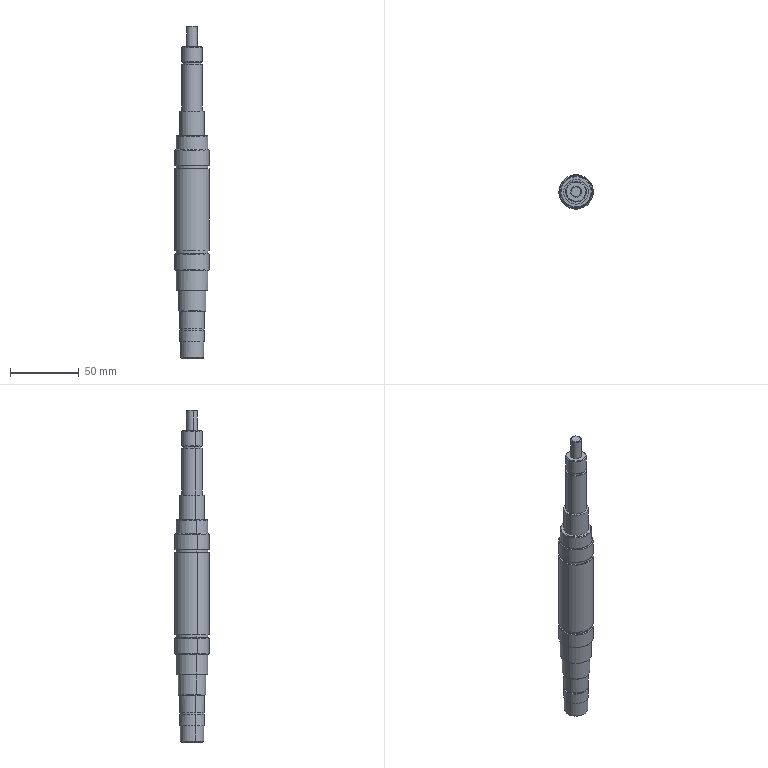Component | SolidWorks | BladeDriveAxis0-2 | 1 solid | 90 faces | box 25 x 25 x 242 mm | volume 78824 mm3 | cylinder 41 | plane 30 | cone 19 | commonest cylinder face diameters 23 x8 18 x6 25 x6 5 x5 15 x4 17 x4 20 x2 13 x2
build123d program:
from build123d import *

# Parameters (mm, degrees)
CUT_EXTRUDE1_2_START = 9.25
CUT_EXTRUDE1_2_DEPTH = 10
CUT_EXTRUDE2_START   = 5.5
CUT_EXTRUDE2_DEPTH   = 10
CUT_EXTRUDE3_START   = 5.8
CUT_EXTRUDE3_DEPTH   = 10
CUT_EXTRUDE1_START   = 9.25
CUT_EXTRUDE1_DEPTH   = 10


with BuildPart() as part:
    # Sketch1_2 → Revolve1 (revolve)
    with BuildSketch(Plane.XY, mode=Mode.PRIVATE) as revolve1_sk:
        Polygon((-96, 8.5), (-96, 9), (-87.7, 9), (-87.7, 8.5), (-86.6, 8.5), (-86.6, 9), (-74, 9), (-74, 9.5), (-73.5, 10), (-59, 10), (-59, 11), (-58.5, 11.5), (-44, 11.5), (-44, 12), (-43.5, 12.5), (-32.5, 12.5), (-32, 12), (-32, 11.5), (-30, 11.5), (-30, 12.5), (30, 12.5), (30, 11.5), (32, 11.5), (32, 12), (32.5, 12.5), (43.5, 12.5), (44, 12), (44, 11.5), (53.5, 11.5), (54, 11), (54, 9), (72, 9), (72, 7.5), (106, 7.5), (106, 6.5), (107.5, 6.5), (107.5, 7), (108, 7.5), (118.5, 7.5), (119, 7), (119, 4), (133.5, 4), (134, 3.5), (134, 0), (-108, 0), (-108, 8), (-107.5, 8.5), align=None)
    revolve(revolve1_sk.sketch.rotate(Axis((-108, 0, 0), (1, 0, 0)), 180), axis=Axis((-108, 0, 0), (1, 0, 0)))

    # Sketch2 → Cut-Extrude1_2 (cut)
    with BuildSketch(Plane(origin=(0, 0, 0), x_dir=(1, 0, 0), z_dir=(0, 1, 0)).offset(CUT_EXTRUDE1_2_START)):
        with BuildLine():
            Line((-44, 2.5), (-32, 2.5))
            ThreePointArc((-32, 2.5), (-29.5, 0), (-32, -2.5))
            Line((-32, -2.5), (-44, -2.5))
            ThreePointArc((-44, -2.5), (-46.5, 0), (-44, 2.5))
        make_face()
        with BuildLine():
            Line((32, 2.5), (44, 2.5))
            ThreePointArc((44, 2.5), (46.5, 0), (44, -2.5))
            Line((44, -2.5), (32, -2.5))
            ThreePointArc((32, -2.5), (29.5, 0), (32, 2.5))
        make_face()
    extrude(amount=CUT_EXTRUDE1_2_DEPTH, mode=Mode.SUBTRACT)

    # Sketch3 → Cut-Extrude2 (cut)
    with BuildSketch(Plane(origin=(0, 0, 0), x_dir=(1, 0, 0), z_dir=(0, 1, 0)).offset(CUT_EXTRUDE2_START)):
        with BuildLine():
            Line((-86.6, 3), (-77, 3))
            ThreePointArc((-77, 3), (-74, 0), (-77, -3))
            Line((-77, -3), (-86.6, -3))
            ThreePointArc((-86.6, -3), (-89.6, 0), (-86.6, 3))
        make_face()
    extrude(amount=CUT_EXTRUDE2_DEPTH, mode=Mode.SUBTRACT)

    # Sketch4 → Cut-Extrude3 (cut)
    with BuildSketch(Plane(origin=(0, 0, 0), x_dir=(1, 0, 0), z_dir=(0, 1, 0)).offset(CUT_EXTRUDE3_START)):
        with BuildLine():
            Line((-108, 2.5), (-99, 2.5))
            ThreePointArc((-99, 2.5), (-96.5, 0), (-99, -2.5))
            Line((-99, -2.5), (-108, -2.5))
            ThreePointArc((-108, -2.5), (-110.5, 0), (-108, 2.5))
        make_face()
    extrude(amount=CUT_EXTRUDE3_DEPTH, mode=Mode.SUBTRACT)

    # Sketch1 → Cut-Extrude1 (cut)
    with BuildSketch(Plane(origin=(0, 0, 0), x_dir=(1, 0, 0), z_dir=(0, 1, 0)).offset(CUT_EXTRUDE1_START)):
        with BuildLine():
            Line((-32, 2.5), (-30, 2.5))
            ThreePointArc((-30, 2.5), (-27.5, 0), (-30, -2.5))
            Line((-30, -2.5), (-32, -2.5))
            ThreePointArc((-32, -2.5), (-34.5, 0), (-32, 2.5))
        make_face()
        with BuildLine():
            Line((30, 2.5), (32, 2.5))
            ThreePointArc((32, 2.5), (34.5, 0), (32, -2.5))
            Line((32, -2.5), (30, -2.5))
            ThreePointArc((30, -2.5), (27.5, 0), (30, 2.5))
        make_face()
    extrude(amount=CUT_EXTRUDE1_DEPTH, mode=Mode.SUBTRACT)


solid = part.part

# Placed as in the assembly
solid = solid.moved(Location((-15.093, -37.782, 235.655), (-90, -17.723, -90)))